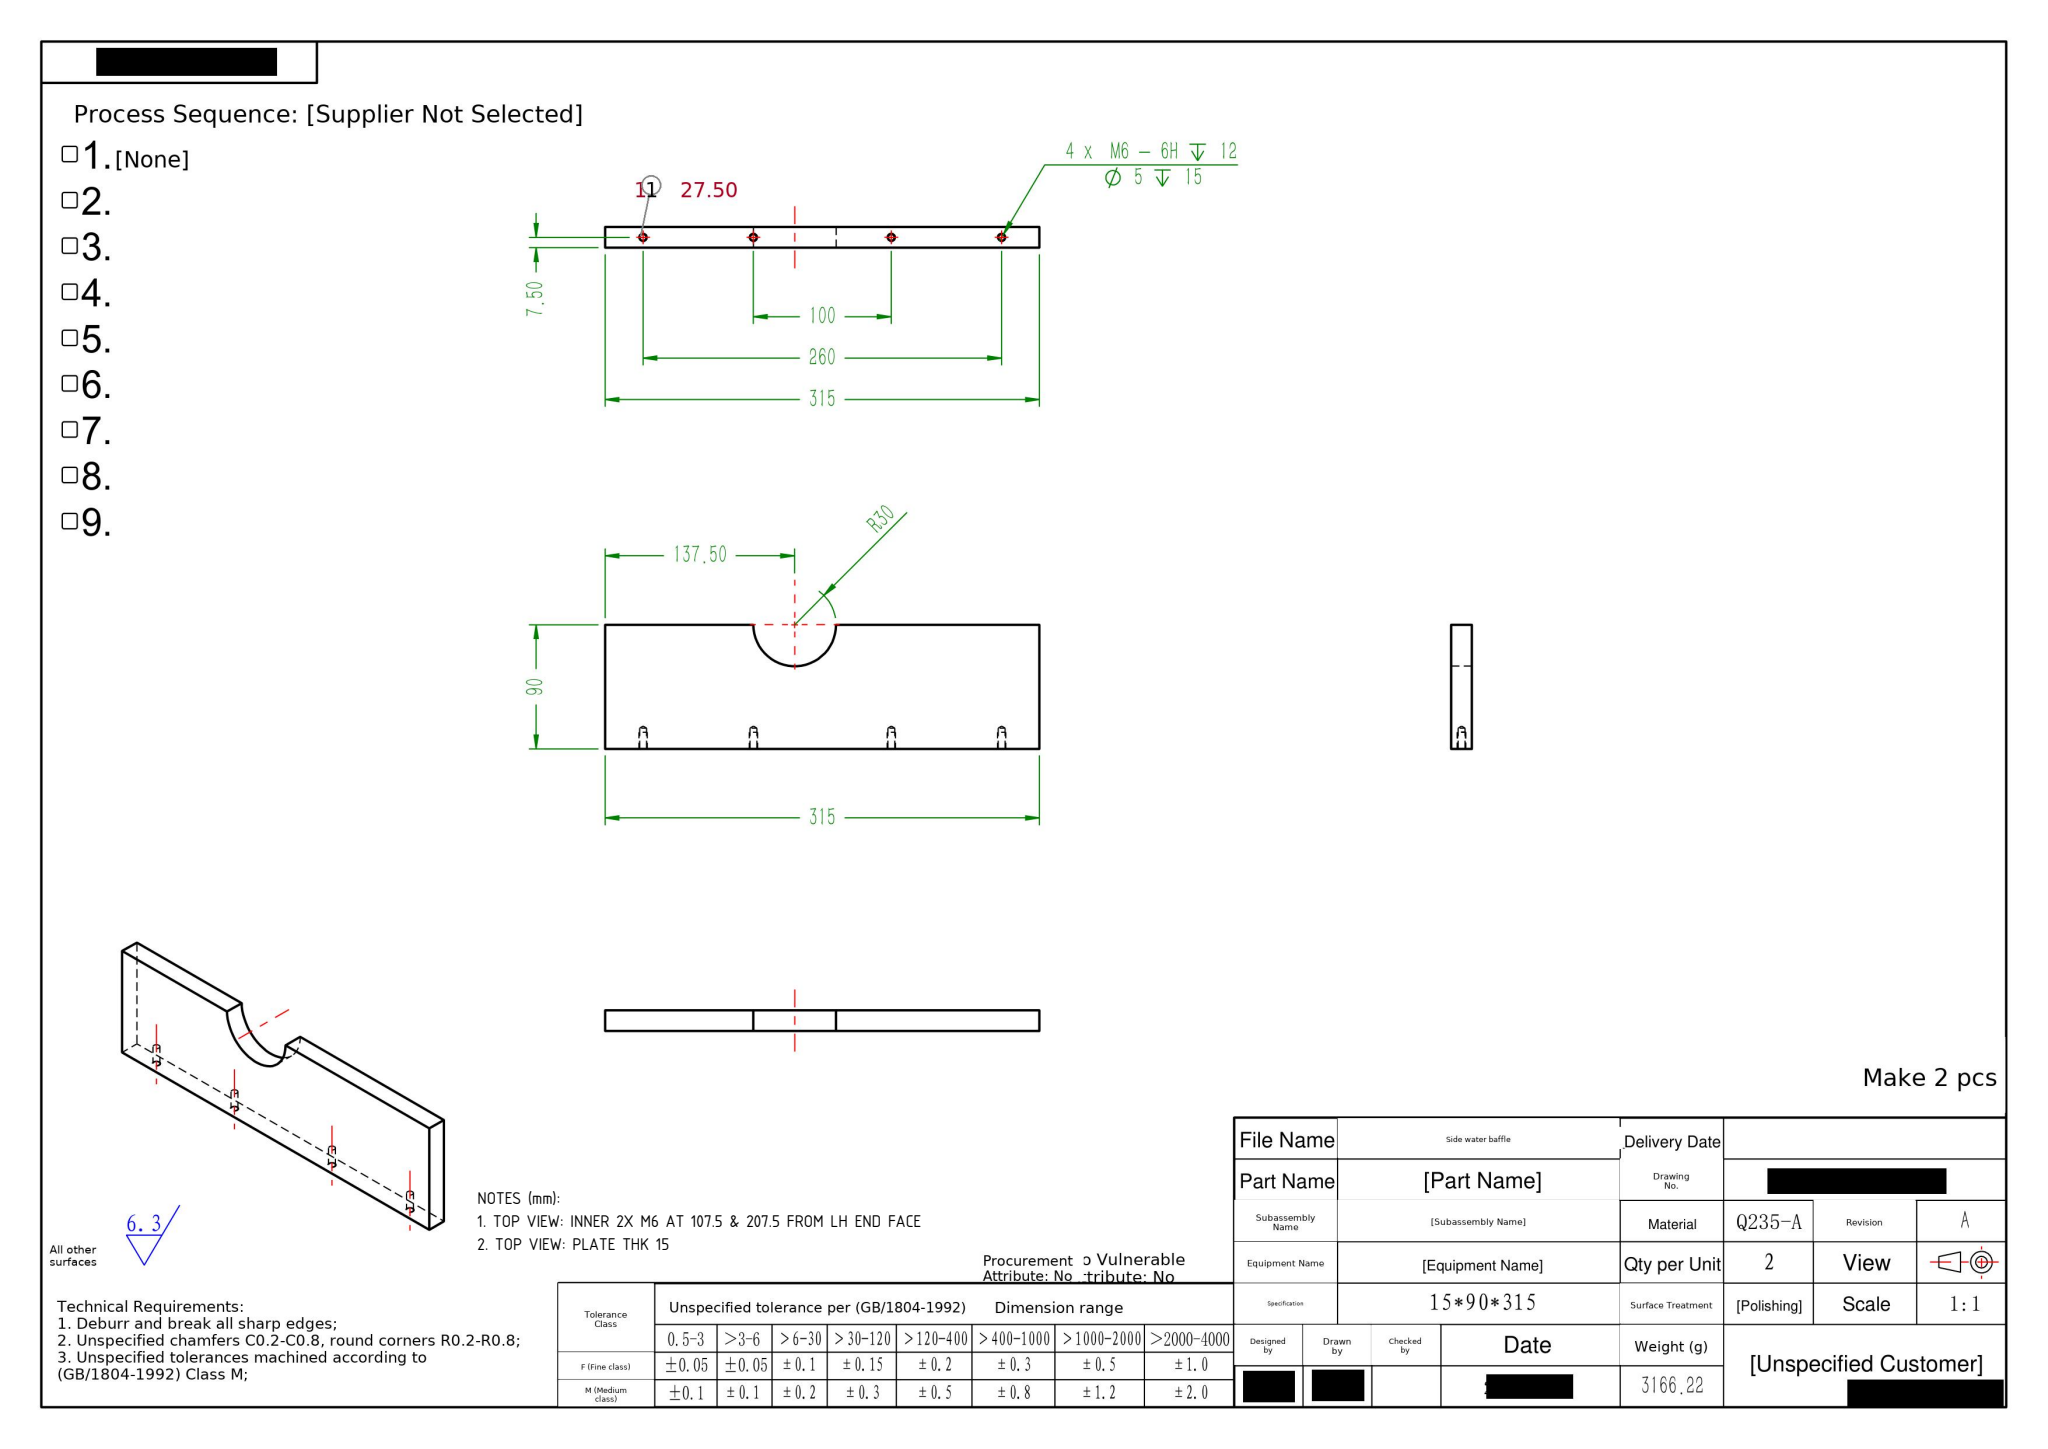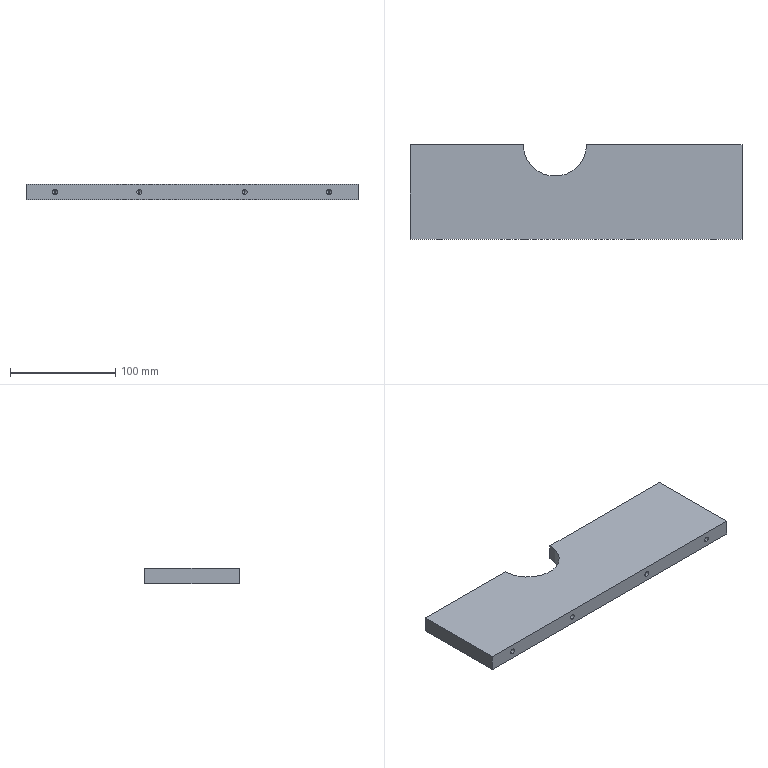Part | SolidWorks | mm | 1 solid | 24 faces | box 315 x 90 x 15 mm | volume 402827 mm3 | cylinder 9 | cone 8 | plane 7 | commonest cylinder face diameters 5 x8 60 x1
Drawing notes:
TOP VIEW: INNER 2X M6 AT 107.5 & 207.5 FROM LH END FACE | from the solid: Ø5 y-axis holes at x=107.5 and x=207.5; x=0 plane is LH end face, bbox 315 long
TOP VIEW: PLATE THK 15 | from the solid: bbox_xyz z=15; planes z=0 and z=15; hole axis at z=7.5
build123d program:
from build123d import *

# Parameters (mm, degrees)
SKETCH1_W             = 315
SKETCH1_H             = 15
BOSS_EXTRUDE1_DEPTH   = 90
SKETCH2_R             = 30
CUT_EXTRUDE1_DEPTH    = 183.02
M6_TAPPED_HOLE1_D     = 5
M6_TAPPED_HOLE1_DEPTH = 15
M6_TAPPED_HOLE1_TIP   = 1.502


with BuildPart() as part:
    # Sketch1 → Boss-Extrude1 (new body)
    with BuildSketch(Plane(origin=(0, 0, 0), x_dir=(1, 0, 0), z_dir=(0, 1, 0))):
        Rectangle(SKETCH1_W, SKETCH1_H)
    extrude(amount=BOSS_EXTRUDE1_DEPTH)

    # Sketch2 → Cut-Extrude1 (cut, through all)
    with BuildSketch(Plane.XY.offset(7.5)):
        with Locations((-20, 90)):
            Circle(SKETCH2_R)
    extrude(amount=-CUT_EXTRUDE1_DEPTH, mode=Mode.SUBTRACT)

    # M6 Tapped Hole1
    with Locations(Plane(origin=(0, 0, 0), x_dir=(-1, 0, 0), z_dir=(0, -1, 0))):
        with Locations((50, 0), (-50, 0), (-130, 0), (130, 0)):
            Hole(M6_TAPPED_HOLE1_D / 2, depth=M6_TAPPED_HOLE1_DEPTH)
            with Locations((0, 0, -(M6_TAPPED_HOLE1_DEPTH + M6_TAPPED_HOLE1_TIP / 2))):  # 118° drill point
                Cone(0, M6_TAPPED_HOLE1_D / 2, M6_TAPPED_HOLE1_TIP, mode=Mode.SUBTRACT)


solid = part.part